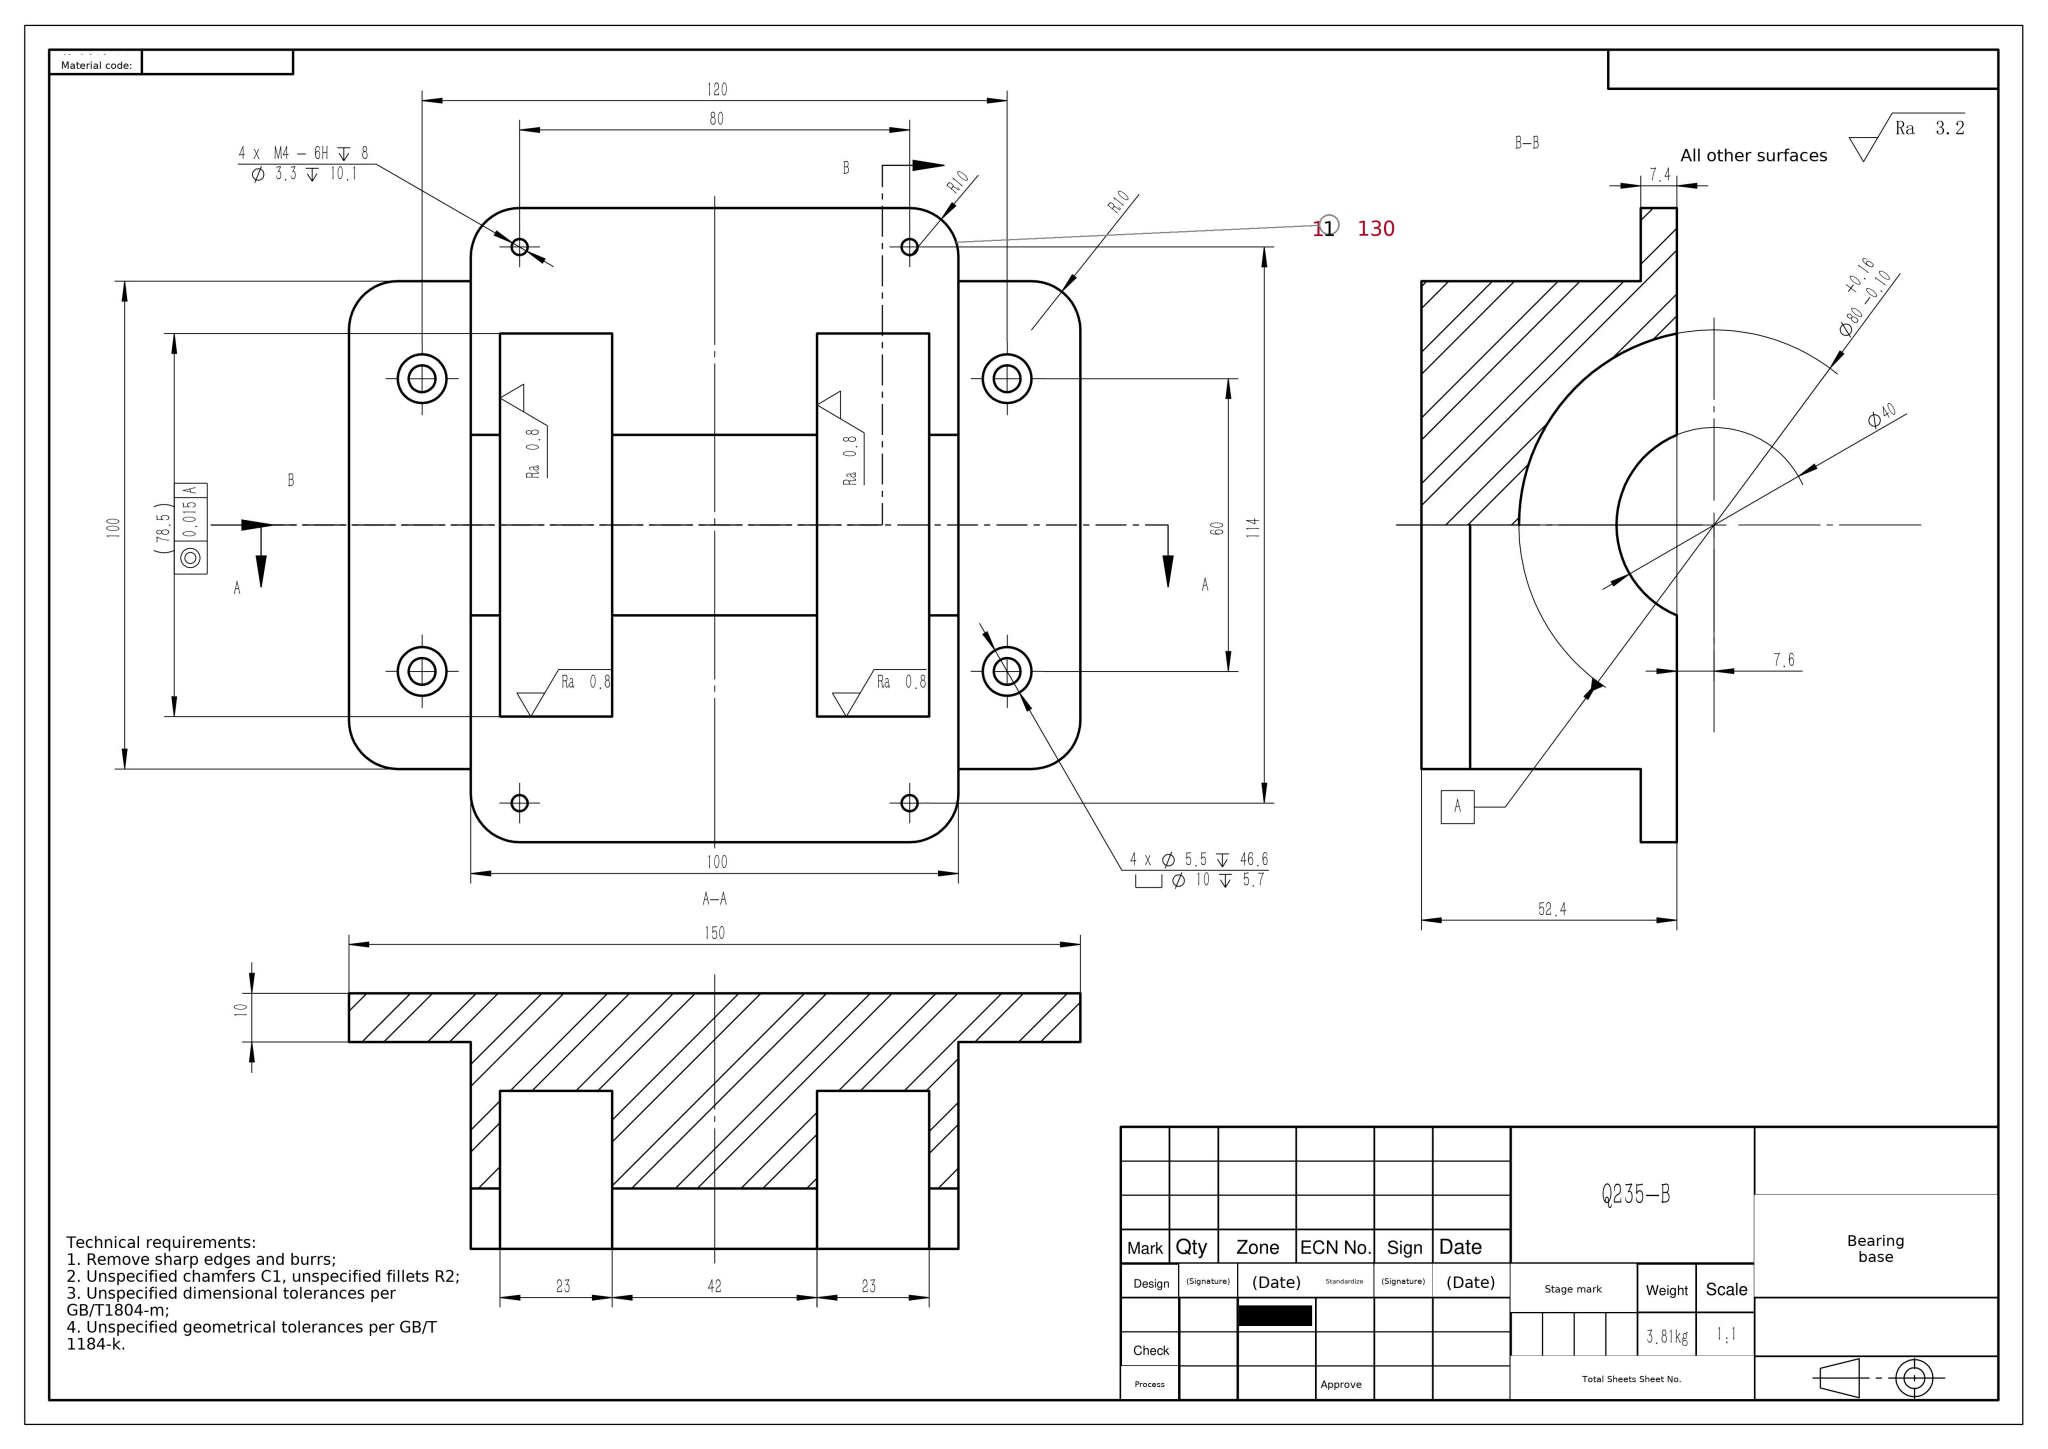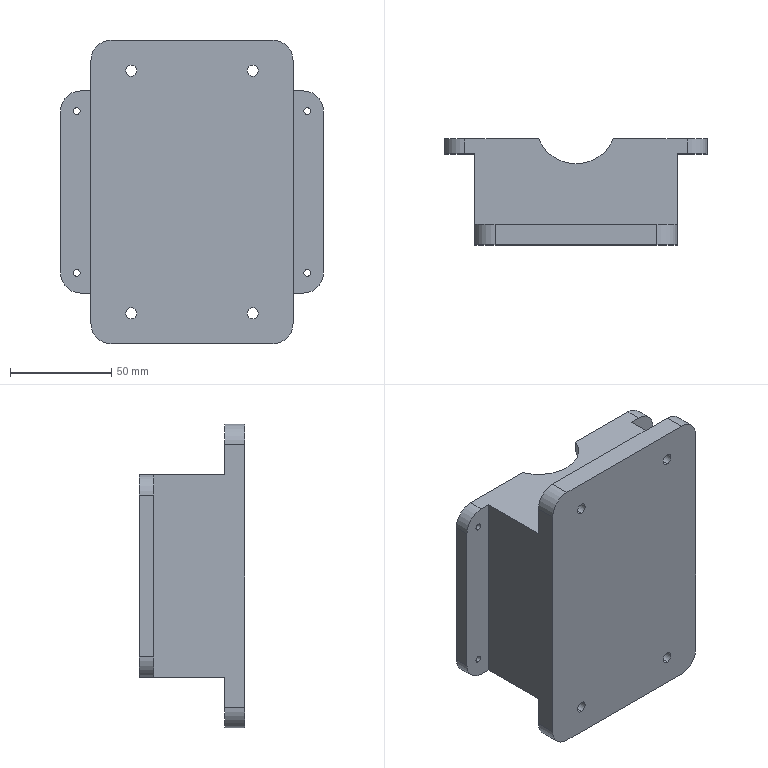Part | SolidWorks | mm | material Q235-B | 1 solid | 60 faces | box 130 x 52.4 x 150 mm | volume 486489 mm3 | cylinder 37 | plane 23 | commonest cylinder face diameters 3.3 x8 10 x8 5.5 x8 20 x8 40 x3 80 x2
build123d program:
from build123d import *

# Parameters (mm, degrees)
SKETCH1_W                                       = 100
SKETCH1_H                                       = 150
BOSS_EXTRUDE1_DEPTH                             = 5
FILLET1_R                                       = 10
BOSS_EXTRUDE3_DEPTH                             = 50
SKETCH5_W                                       = 130
SKETCH5_H                                       = 15
BOSS_EXTRUDE4_DEPTH                             = 100
CUT_EXTRUDE2_DEPTH                              = 15
FILLET3_R                                       = 10
SKETCH6_R                                       = 20
CUT_EXTRUDE3_DEPTH                              = 176.713
CUT_EXTRUDE4_START                              = -6
SKETCH7_R                                       = 40
CUT_EXTRUDE4_DEPTH                              = 23
FILLET6_R                                       = 5
SKETCH11_W                                      = 281.527
SKETCH11_H                                      = 90.878
CUT_EXTRUDE5_DEPTH                              = 176.713
M5_HEX_SOCKET_HEAD_CAP_SCREW_CBORE1_D           = 5.5
M5_HEX_SOCKET_HEAD_CAP_SCREW_CBORE1_DEPTH       = 46.55
M5_HEX_SOCKET_HEAD_CAP_SCREW_CBORE1_CBORE_D     = 10
M5_HEX_SOCKET_HEAD_CAP_SCREW_CBORE1_CBORE_DEPTH = 5.7
M5_HEX_SOCKET_HEAD_CAP_SCREW_CBORE1_TIP         = 1.652
M4_TAPPED_HOLE1_D                               = 3.3
M4_TAPPED_HOLE1_DEPTH                           = 10.1
M4_TAPPED_HOLE1_TIP                             = 0.9914
FILLET7_R                                       = 10


with BuildPart() as part:
    # Sketch1 → Boss-Extrude1 (new, symmetric)
    with BuildSketch(Plane(origin=(0, 0, 0), x_dir=(1, 0, 0), z_dir=(0, 1, 0))):
        Rectangle(SKETCH1_W, SKETCH1_H)
    extrude(amount=BOSS_EXTRUDE1_DEPTH, both=True)

    # Fillet1
    fillet1_edges = [part.edges().sort_by_distance(p)[0] for p in [
        (50, 0, 75),
        (-50, 0, 75),
        (-50, 0, -75),
        (50, 0, -75),
    ]]
    fillet(fillet1_edges, radius=FILLET1_R)

    # Sketch3 → Boss-Extrude3 (add, symmetric)
    with BuildSketch(Plane.XY):
        with BuildLine():
            Line((-50, 25), (-50, 5))
            Line((-50, 5), (50, 5))
            Line((50, 5), (50, 25))
            Line((50, 25), (50, 55))
            ThreePointArc((50, 55), (0, 105), (-50, 55))
            Line((-50, 55), (-50, 25))
        make_face()
    extrude(amount=BOSS_EXTRUDE3_DEPTH, both=True)

    # Sketch5 → Boss-Extrude4 (add)
    with BuildSketch(Plane.XY.offset(50)):
        with Locations((0, 47.5)):
            Rectangle(SKETCH5_W, SKETCH5_H)
    extrude(amount=-BOSS_EXTRUDE4_DEPTH)

    # Sketch4 → Cut-Extrude2 (cut, symmetric)
    with BuildSketch(Plane.XY):
        with BuildLine():
            Line((22.5, 55), (50, 55))
            ThreePointArc((50, 55), (0, 105), (-50, 55))
            Line((-50, 55), (-22.5, 55))
            ThreePointArc((-22.5, 55), (0, 77.5), (22.5, 55))
        make_face()
    extrude(amount=CUT_EXTRUDE2_DEPTH, both=True, mode=Mode.SUBTRACT)

    # Fillet3
    fillet3_edges = [part.edges().sort_by_distance(p)[0] for p in [
        (0, 105, -15),
        (0, 105, 15),
    ]]
    fillet(fillet3_edges, radius=FILLET3_R)

    # Sketch6 → Cut-Extrude3 (cut, through all)
    with BuildSketch(Plane.XY.offset(50)):
        with Locations((0, 55)):
            Circle(SKETCH6_R)
    extrude(amount=-CUT_EXTRUDE3_DEPTH, mode=Mode.SUBTRACT)

    # Sketch7 → Cut-Extrude4 (cut)
    with BuildSketch(Plane.XY.offset(50).offset(CUT_EXTRUDE4_START)):
        with Locations((0, 55)):
            Circle(SKETCH7_R)
    cut_extrude4 = extrude(amount=-CUT_EXTRUDE4_DEPTH, mode=Mode.SUBTRACT)

    # Mirror1: Cut-Extrude4 across plane
    add(cut_extrude4.mirror(Plane.XY), mode=Mode.SUBTRACT)

    # Fillet6
    fillet6_edges = [part.edges().sort_by_distance(p)[0] for p in [
        (0, 105, -50),
        (0, 105, 50),
    ]]
    fillet(fillet6_edges, radius=FILLET6_R)

    # Sketch11 → Cut-Extrude5 (cut, through all)
    with BuildSketch(Plane(origin=(0, 0, -50), x_dir=(-1, 0, 0), z_dir=(0, 0, -1))):
        with Locations((-30.758, 92.834)):
            Rectangle(SKETCH11_W, SKETCH11_H)
    extrude(amount=-CUT_EXTRUDE5_DEPTH, mode=Mode.SUBTRACT)

    # M5 Hex Socket Head Cap Screw CBORE1
    with Locations(Plane(origin=(0, 5, 0), x_dir=(1, 0, 0), z_dir=(0, 1, 0))):
        with Locations((-30, 60), (30, 60), (30, -60), (-30, -60)):
            CounterBoreHole(M5_HEX_SOCKET_HEAD_CAP_SCREW_CBORE1_D / 2, M5_HEX_SOCKET_HEAD_CAP_SCREW_CBORE1_CBORE_D / 2, M5_HEX_SOCKET_HEAD_CAP_SCREW_CBORE1_CBORE_DEPTH, depth=M5_HEX_SOCKET_HEAD_CAP_SCREW_CBORE1_DEPTH)
            with Locations((0, 0, -(M5_HEX_SOCKET_HEAD_CAP_SCREW_CBORE1_DEPTH + M5_HEX_SOCKET_HEAD_CAP_SCREW_CBORE1_TIP / 2))):  # 118° drill point
                Cone(0, M5_HEX_SOCKET_HEAD_CAP_SCREW_CBORE1_D / 2, M5_HEX_SOCKET_HEAD_CAP_SCREW_CBORE1_TIP, mode=Mode.SUBTRACT)

    # M4 Tapped Hole1
    with Locations(Plane(origin=(0, 47.395, 0), x_dir=(1, 0, 0), z_dir=(0, 1, 0))):
        with Locations((-57, 40), (-57, -40), (57, -40), (57, 40)):
            Hole(M4_TAPPED_HOLE1_D / 2, depth=M4_TAPPED_HOLE1_DEPTH)
            with Locations((0, 0, -(M4_TAPPED_HOLE1_DEPTH + M4_TAPPED_HOLE1_TIP / 2))):  # 118° drill point
                Cone(0, M4_TAPPED_HOLE1_D / 2, M4_TAPPED_HOLE1_TIP, mode=Mode.SUBTRACT)

    # Fillet7
    fillet7_edges = [part.edges().sort_by_distance(p)[0] for p in [
        (65, 43.698, -50),
        (-65, 43.698, 50),
        (65, 43.698, 50),
        (-65, 43.698, -50),
    ]]
    fillet(fillet7_edges, radius=FILLET7_R)


solid = part.part